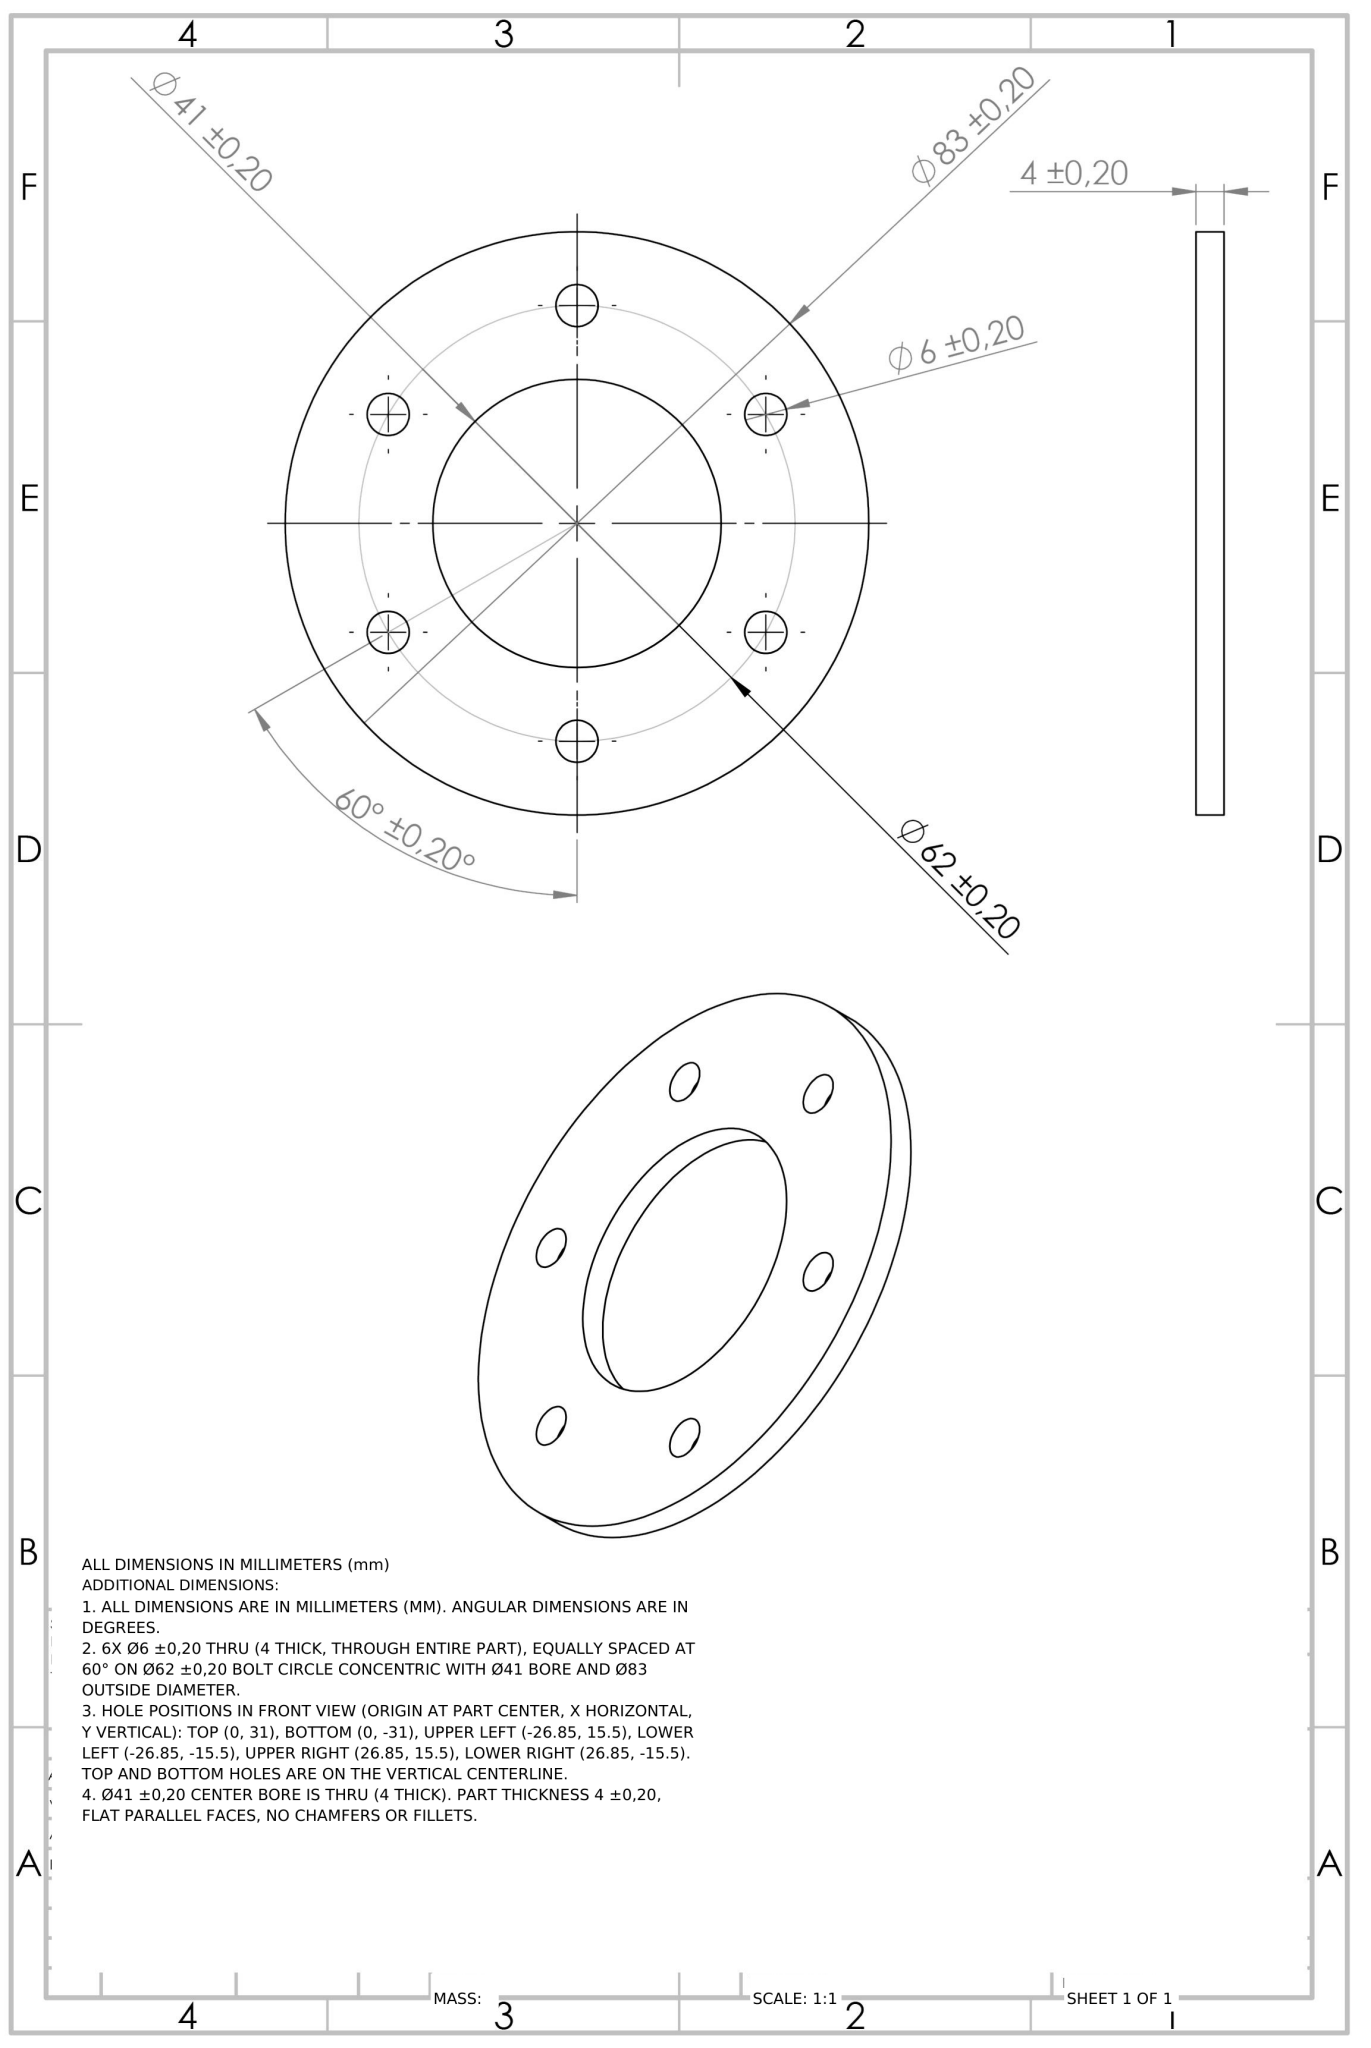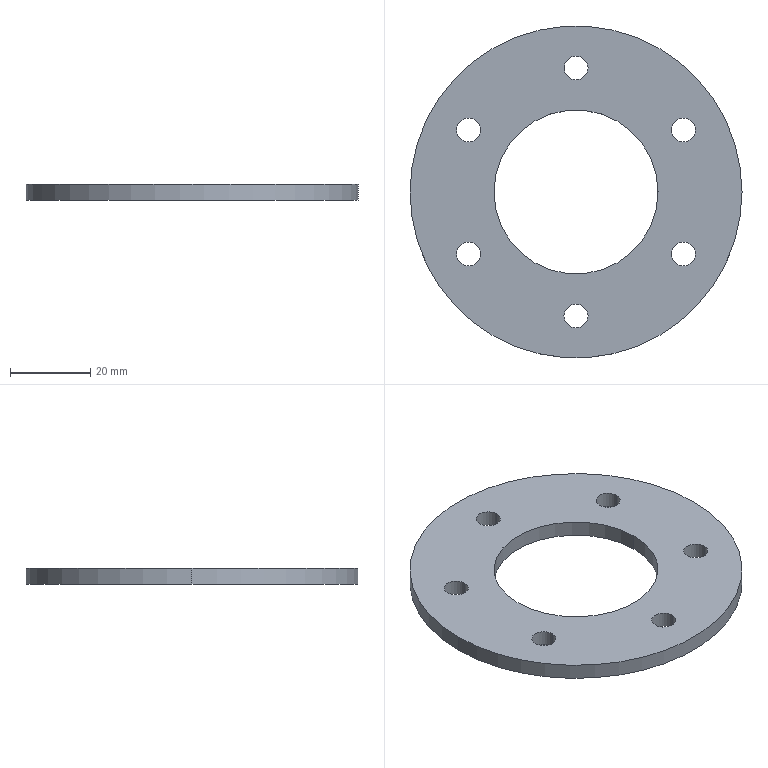Part | NX | mm | Six-Bolt Circular Flange Plate | 1 solid | 18 faces | box 83 x 83 x 4 mm | volume 15683 mm3 | cylinder 16 | plane 2 | commonest cylinder face diameters 6 x12 41 x2 83 x2
STEP:
#1=COLOUR_RGB('',0.7922,0.8196,0.9333);
#2=FILL_AREA_STYLE_COLOUR('',#1);
#3=FILL_AREA_STYLE('',(#2));
#4=SURFACE_STYLE_FILL_AREA(#3);
#5=SURFACE_SIDE_STYLE('',(#4));
#6=SURFACE_STYLE_USAGE(.BOTH.,#5);
#7=PRESENTATION_STYLE_ASSIGNMENT((#6));
#8=CARTESIAN_POINT('',(-29.847,15.5,4.));
#9=VERTEX_POINT('',#8);
#10=CARTESIAN_POINT('',(-23.847,15.5,4.));
#11=VERTEX_POINT('',#10);
#12=CARTESIAN_POINT('',(-26.847,15.5,4.));
#13=DIRECTION('',(0.,0.,1.));
#14=DIRECTION('',(1.,0.,0.));
#15=AXIS2_PLACEMENT_3D('',#12,#13,#14);
#16=CIRCLE('',#15,3.);
#17=EDGE_CURVE('',#9,#11,#16,.T.);
#18=ORIENTED_EDGE('',*,*,#17,.T.);
#19=CARTESIAN_POINT('',(-23.847,15.5,0.));
#20=VERTEX_POINT('',#19);
#21=CARTESIAN_POINT('',(-23.847,15.5,4.));
#22=DIRECTION('',(0.,0.,-1.));
#23=VECTOR('',#22,1000.);
#24=LINE('',#21,#23);
#25=EDGE_CURVE('',#11,#20,#24,.T.);
#26=ORIENTED_EDGE('',*,*,#25,.T.);
#27=CARTESIAN_POINT('',(-29.847,15.5,0.));
#28=VERTEX_POINT('',#27);
#29=CARTESIAN_POINT('',(-26.847,15.5,0.));
#30=DIRECTION('',(0.,0.,1.));
#31=DIRECTION('',(1.,0.,0.));
#32=AXIS2_PLACEMENT_3D('',#29,#30,#31);
#33=CIRCLE('',#32,3.);
#34=EDGE_CURVE('',#28,#20,#33,.T.);
#35=ORIENTED_EDGE('',*,*,#34,.F.);
#36=CARTESIAN_POINT('',(-29.847,15.5,4.));
#37=DIRECTION('',(0.,0.,-1.));
#38=VECTOR('',#37,1000.);
#39=LINE('',#36,#38);
#40=EDGE_CURVE('',#9,#28,#39,.T.);
#41=ORIENTED_EDGE('',*,*,#40,.F.);
#42=EDGE_LOOP('',(#18,#26,#35,#41));
#43=FACE_OUTER_BOUND('',#42,.T.);
#44=CARTESIAN_POINT('',(-26.847,15.5,4.));
#45=DIRECTION('',(0.,0.,-1.));
#46=DIRECTION('',(-1.,0.,0.));
#47=AXIS2_PLACEMENT_3D('',#44,#45,#46);
#48=CYLINDRICAL_SURFACE('',#47,3.);
#49=ADVANCED_FACE('',(#43),#48,.F.);
#50=CARTESIAN_POINT('',(-29.847,-15.5,4.));
#51=VERTEX_POINT('',#50);
#52=CARTESIAN_POINT('',(-23.847,-15.5,4.));
#53=VERTEX_POINT('',#52);
#54=CARTESIAN_POINT('',(-26.847,-15.5,4.));
#55=DIRECTION('',(0.,0.,1.));
#56=DIRECTION('',(1.,0.,0.));
#57=AXIS2_PLACEMENT_3D('',#54,#55,#56);
#58=CIRCLE('',#57,3.);
#59=EDGE_CURVE('',#51,#53,#58,.T.);
#60=ORIENTED_EDGE('',*,*,#59,.T.);
#61=CARTESIAN_POINT('',(-23.847,-15.5,0.));
#62=VERTEX_POINT('',#61);
#63=CARTESIAN_POINT('',(-23.847,-15.5,4.));
#64=DIRECTION('',(0.,0.,-1.));
#65=VECTOR('',#64,1000.);
#66=LINE('',#63,#65);
#67=EDGE_CURVE('',#53,#62,#66,.T.);
#68=ORIENTED_EDGE('',*,*,#67,.T.);
#69=CARTESIAN_POINT('',(-29.847,-15.5,0.));
#70=VERTEX_POINT('',#69);
#71=CARTESIAN_POINT('',(-26.847,-15.5,0.));
#72=DIRECTION('',(0.,0.,1.));
#73=DIRECTION('',(1.,0.,0.));
#74=AXIS2_PLACEMENT_3D('',#71,#72,#73);
#75=CIRCLE('',#74,3.);
#76=EDGE_CURVE('',#70,#62,#75,.T.);
#77=ORIENTED_EDGE('',*,*,#76,.F.);
#78=CARTESIAN_POINT('',(-29.847,-15.5,4.));
#79=DIRECTION('',(0.,0.,-1.));
#80=VECTOR('',#79,1000.);
#81=LINE('',#78,#80);
#82=EDGE_CURVE('',#51,#70,#81,.T.);
#83=ORIENTED_EDGE('',*,*,#82,.F.);
#84=EDGE_LOOP('',(#60,#68,#77,#83));
#85=FACE_OUTER_BOUND('',#84,.T.);
#86=CARTESIAN_POINT('',(-26.847,-15.5,4.));
#87=DIRECTION('',(0.,0.,-1.));
#88=DIRECTION('',(-1.,0.,0.));
#89=AXIS2_PLACEMENT_3D('',#86,#87,#88);
#90=CYLINDRICAL_SURFACE('',#89,3.);
#91=ADVANCED_FACE('',(#85),#90,.F.);
#92=CARTESIAN_POINT('',(-3.,-31.,4.));
#93=VERTEX_POINT('',#92);
#94=CARTESIAN_POINT('',(3.,-31.,4.));
#95=VERTEX_POINT('',#94);
#96=CARTESIAN_POINT('',(0.,-31.,4.));
#97=DIRECTION('',(0.,0.,1.));
#98=DIRECTION('',(1.,0.,0.));
#99=AXIS2_PLACEMENT_3D('',#96,#97,#98);
#100=CIRCLE('',#99,3.);
#101=EDGE_CURVE('',#93,#95,#100,.T.);
#102=ORIENTED_EDGE('',*,*,#101,.T.);
#103=CARTESIAN_POINT('',(3.,-31.,0.));
#104=VERTEX_POINT('',#103);
#105=CARTESIAN_POINT('',(3.,-31.,4.));
#106=DIRECTION('',(0.,0.,-1.));
#107=VECTOR('',#106,1000.);
#108=LINE('',#105,#107);
#109=EDGE_CURVE('',#95,#104,#108,.T.);
#110=ORIENTED_EDGE('',*,*,#109,.T.);
#111=CARTESIAN_POINT('',(-3.,-31.,0.));
#112=VERTEX_POINT('',#111);
#113=CARTESIAN_POINT('',(0.,-31.,0.));
#114=DIRECTION('',(0.,0.,1.));
#115=DIRECTION('',(1.,0.,0.));
#116=AXIS2_PLACEMENT_3D('',#113,#114,#115);
#117=CIRCLE('',#116,3.);
#118=EDGE_CURVE('',#112,#104,#117,.T.);
#119=ORIENTED_EDGE('',*,*,#118,.F.);
#120=CARTESIAN_POINT('',(-3.,-31.,4.));
#121=DIRECTION('',(0.,0.,-1.));
#122=VECTOR('',#121,1000.);
#123=LINE('',#120,#122);
#124=EDGE_CURVE('',#93,#112,#123,.T.);
#125=ORIENTED_EDGE('',*,*,#124,.F.);
#126=EDGE_LOOP('',(#102,#110,#119,#125));
#127=FACE_OUTER_BOUND('',#126,.T.);
#128=CARTESIAN_POINT('',(0.,-31.,4.));
#129=DIRECTION('',(0.,0.,-1.));
#130=DIRECTION('',(-1.,0.,0.));
#131=AXIS2_PLACEMENT_3D('',#128,#129,#130);
#132=CYLINDRICAL_SURFACE('',#131,3.);
#133=ADVANCED_FACE('',(#127),#132,.F.);
#134=CARTESIAN_POINT('',(23.847,-15.5,4.));
#135=VERTEX_POINT('',#134);
#136=CARTESIAN_POINT('',(29.847,-15.5,4.));
#137=VERTEX_POINT('',#136);
#138=CARTESIAN_POINT('',(26.847,-15.5,4.));
#139=DIRECTION('',(0.,0.,1.));
#140=DIRECTION('',(1.,0.,0.));
#141=AXIS2_PLACEMENT_3D('',#138,#139,#140);
#142=CIRCLE('',#141,3.);
#143=EDGE_CURVE('',#135,#137,#142,.T.);
#144=ORIENTED_EDGE('',*,*,#143,.T.);
#145=CARTESIAN_POINT('',(29.847,-15.5,0.));
#146=VERTEX_POINT('',#145);
#147=CARTESIAN_POINT('',(29.847,-15.5,4.));
#148=DIRECTION('',(0.,0.,-1.));
#149=VECTOR('',#148,1000.);
#150=LINE('',#147,#149);
#151=EDGE_CURVE('',#137,#146,#150,.T.);
#152=ORIENTED_EDGE('',*,*,#151,.T.);
#153=CARTESIAN_POINT('',(23.847,-15.5,0.));
#154=VERTEX_POINT('',#153);
#155=CARTESIAN_POINT('',(26.847,-15.5,0.));
#156=DIRECTION('',(0.,0.,1.));
#157=DIRECTION('',(1.,0.,0.));
#158=AXIS2_PLACEMENT_3D('',#155,#156,#157);
#159=CIRCLE('',#158,3.);
#160=EDGE_CURVE('',#154,#146,#159,.T.);
#161=ORIENTED_EDGE('',*,*,#160,.F.);
#162=CARTESIAN_POINT('',(23.847,-15.5,4.));
#163=DIRECTION('',(0.,0.,-1.));
#164=VECTOR('',#163,1000.);
#165=LINE('',#162,#164);
#166=EDGE_CURVE('',#135,#154,#165,.T.);
#167=ORIENTED_EDGE('',*,*,#166,.F.);
#168=EDGE_LOOP('',(#144,#152,#161,#167));
#169=FACE_OUTER_BOUND('',#168,.T.);
#170=CARTESIAN_POINT('',(26.847,-15.5,4.));
#171=DIRECTION('',(0.,0.,-1.));
#172=DIRECTION('',(-1.,0.,0.));
#173=AXIS2_PLACEMENT_3D('',#170,#171,#172);
#174=CYLINDRICAL_SURFACE('',#173,3.);
#175=ADVANCED_FACE('',(#169),#174,.F.);
#176=CARTESIAN_POINT('',(23.847,15.5,4.));
#177=VERTEX_POINT('',#176);
#178=CARTESIAN_POINT('',(29.847,15.5,4.));
#179=VERTEX_POINT('',#178);
#180=CARTESIAN_POINT('',(26.847,15.5,4.));
#181=DIRECTION('',(0.,0.,1.));
#182=DIRECTION('',(1.,0.,0.));
#183=AXIS2_PLACEMENT_3D('',#180,#181,#182);
#184=CIRCLE('',#183,3.);
#185=EDGE_CURVE('',#177,#179,#184,.T.);
#186=ORIENTED_EDGE('',*,*,#185,.T.);
#187=CARTESIAN_POINT('',(29.847,15.5,0.));
#188=VERTEX_POINT('',#187);
#189=CARTESIAN_POINT('',(29.847,15.5,4.));
#190=DIRECTION('',(0.,0.,-1.));
#191=VECTOR('',#190,1000.);
#192=LINE('',#189,#191);
#193=EDGE_CURVE('',#179,#188,#192,.T.);
#194=ORIENTED_EDGE('',*,*,#193,.T.);
#195=CARTESIAN_POINT('',(23.847,15.5,0.));
#196=VERTEX_POINT('',#195);
#197=CARTESIAN_POINT('',(26.847,15.5,0.));
#198=DIRECTION('',(0.,0.,1.));
#199=DIRECTION('',(1.,0.,0.));
#200=AXIS2_PLACEMENT_3D('',#197,#198,#199);
#201=CIRCLE('',#200,3.);
#202=EDGE_CURVE('',#196,#188,#201,.T.);
#203=ORIENTED_EDGE('',*,*,#202,.F.);
#204=CARTESIAN_POINT('',(23.847,15.5,4.));
#205=DIRECTION('',(0.,0.,-1.));
#206=VECTOR('',#205,1000.);
#207=LINE('',#204,#206);
#208=EDGE_CURVE('',#177,#196,#207,.T.);
#209=ORIENTED_EDGE('',*,*,#208,.F.);
#210=EDGE_LOOP('',(#186,#194,#203,#209));
#211=FACE_OUTER_BOUND('',#210,.T.);
#212=CARTESIAN_POINT('',(26.847,15.5,4.));
#213=DIRECTION('',(0.,0.,-1.));
#214=DIRECTION('',(-1.,0.,0.));
#215=AXIS2_PLACEMENT_3D('',#212,#213,#214);
#216=CYLINDRICAL_SURFACE('',#215,3.);
#217=ADVANCED_FACE('',(#211),#216,.F.);
#218=CARTESIAN_POINT('',(-3.,31.,4.));
#219=VERTEX_POINT('',#218);
#220=CARTESIAN_POINT('',(3.,31.,4.));
#221=VERTEX_POINT('',#220);
#222=CARTESIAN_POINT('',(0.,31.,4.));
#223=DIRECTION('',(0.,0.,1.));
#224=DIRECTION('',(1.,0.,0.));
#225=AXIS2_PLACEMENT_3D('',#222,#223,#224);
#226=CIRCLE('',#225,3.);
#227=EDGE_CURVE('',#219,#221,#226,.T.);
#228=ORIENTED_EDGE('',*,*,#227,.T.);
#229=CARTESIAN_POINT('',(3.,31.,0.));
#230=VERTEX_POINT('',#229);
#231=CARTESIAN_POINT('',(3.,31.,4.));
#232=DIRECTION('',(0.,0.,-1.));
#233=VECTOR('',#232,1000.);
#234=LINE('',#231,#233);
#235=EDGE_CURVE('',#221,#230,#234,.T.);
#236=ORIENTED_EDGE('',*,*,#235,.T.);
#237=CARTESIAN_POINT('',(-3.,31.,0.));
#238=VERTEX_POINT('',#237);
#239=CARTESIAN_POINT('',(0.,31.,0.));
#240=DIRECTION('',(0.,0.,1.));
#241=DIRECTION('',(1.,0.,0.));
#242=AXIS2_PLACEMENT_3D('',#239,#240,#241);
#243=CIRCLE('',#242,3.);
#244=EDGE_CURVE('',#238,#230,#243,.T.);
#245=ORIENTED_EDGE('',*,*,#244,.F.);
#246=CARTESIAN_POINT('',(-3.,31.,4.));
#247=DIRECTION('',(0.,0.,-1.));
#248=VECTOR('',#247,1000.);
#249=LINE('',#246,#248);
#250=EDGE_CURVE('',#219,#238,#249,.T.);
#251=ORIENTED_EDGE('',*,*,#250,.F.);
#252=EDGE_LOOP('',(#228,#236,#245,#251));
#253=FACE_OUTER_BOUND('',#252,.T.);
#254=CARTESIAN_POINT('',(0.,31.,4.));
#255=DIRECTION('',(0.,0.,-1.));
#256=DIRECTION('',(-1.,0.,0.));
#257=AXIS2_PLACEMENT_3D('',#254,#255,#256);
#258=CYLINDRICAL_SURFACE('',#257,3.);
#259=ADVANCED_FACE('',(#253),#258,.F.);
#260=CARTESIAN_POINT('',(-20.5,0.,4.));
#261=VERTEX_POINT('',#260);
#262=CARTESIAN_POINT('',(20.5,0.,4.));
#263=VERTEX_POINT('',#262);
#264=CARTESIAN_POINT('',(0.,0.,4.));
#265=DIRECTION('',(0.,0.,1.));
#266=DIRECTION('',(1.,0.,0.));
#267=AXIS2_PLACEMENT_3D('',#264,#265,#266);
#268=CIRCLE('',#267,20.5);
#269=EDGE_CURVE('',#261,#263,#268,.T.);
#270=ORIENTED_EDGE('',*,*,#269,.T.);
#271=CARTESIAN_POINT('',(20.5,0.,0.));
#272=VERTEX_POINT('',#271);
#273=CARTESIAN_POINT('',(20.5,0.,4.));
#274=DIRECTION('',(0.,0.,-1.));
#275=VECTOR('',#274,1000.);
#276=LINE('',#273,#275);
#277=EDGE_CURVE('',#263,#272,#276,.T.);
#278=ORIENTED_EDGE('',*,*,#277,.T.);
#279=CARTESIAN_POINT('',(-20.5,0.,0.));
#280=VERTEX_POINT('',#279);
#281=CARTESIAN_POINT('',(0.,0.,0.));
#282=DIRECTION('',(0.,0.,1.));
#283=DIRECTION('',(1.,0.,0.));
#284=AXIS2_PLACEMENT_3D('',#281,#282,#283);
#285=CIRCLE('',#284,20.5);
#286=EDGE_CURVE('',#280,#272,#285,.T.);
#287=ORIENTED_EDGE('',*,*,#286,.F.);
#288=CARTESIAN_POINT('',(-20.5,0.,4.));
#289=DIRECTION('',(0.,0.,-1.));
#290=VECTOR('',#289,1000.);
#291=LINE('',#288,#290);
#292=EDGE_CURVE('',#261,#280,#291,.T.);
#293=ORIENTED_EDGE('',*,*,#292,.F.);
#294=EDGE_LOOP('',(#270,#278,#287,#293));
#295=FACE_OUTER_BOUND('',#294,.T.);
#296=CARTESIAN_POINT('',(0.,0.,4.));
#297=DIRECTION('',(0.,0.,-1.));
#298=DIRECTION('',(-1.,0.,0.));
#299=AXIS2_PLACEMENT_3D('',#296,#297,#298);
#300=CYLINDRICAL_SURFACE('',#299,20.5);
#301=ADVANCED_FACE('',(#295),#300,.F.);
#302=CARTESIAN_POINT('',(41.5,0.,4.));
#303=VERTEX_POINT('',#302);
#304=CARTESIAN_POINT('',(-41.5,0.,4.));
#305=VERTEX_POINT('',#304);
#306=CARTESIAN_POINT('',(0.,0.,4.));
#307=DIRECTION('',(0.,0.,1.));
#308=DIRECTION('',(1.,0.,0.));
#309=AXIS2_PLACEMENT_3D('',#306,#307,#308);
#310=CIRCLE('',#309,41.5);
#311=EDGE_CURVE('',#303,#305,#310,.T.);
#312=ORIENTED_EDGE('',*,*,#311,.F.);
#313=CARTESIAN_POINT('',(41.5,0.,0.));
#314=VERTEX_POINT('',#313);
#315=CARTESIAN_POINT('',(41.5,0.,4.));
#316=DIRECTION('',(0.,0.,-1.));
#317=VECTOR('',#316,1000.);
#318=LINE('',#315,#317);
#319=EDGE_CURVE('',#303,#314,#318,.T.);
#320=ORIENTED_EDGE('',*,*,#319,.T.);
#321=CARTESIAN_POINT('',(-41.5,0.,0.));
#322=VERTEX_POINT('',#321);
#323=CARTESIAN_POINT('',(0.,0.,0.));
#324=DIRECTION('',(0.,0.,1.));
#325=DIRECTION('',(1.,0.,0.));
#326=AXIS2_PLACEMENT_3D('',#323,#324,#325);
#327=CIRCLE('',#326,41.5);
#328=EDGE_CURVE('',#314,#322,#327,.T.);
#329=ORIENTED_EDGE('',*,*,#328,.T.);
#330=CARTESIAN_POINT('',(-41.5,0.,4.));
#331=DIRECTION('',(0.,0.,-1.));
#332=VECTOR('',#331,1000.);
#333=LINE('',#330,#332);
#334=EDGE_CURVE('',#305,#322,#333,.T.);
#335=ORIENTED_EDGE('',*,*,#334,.F.);
#336=EDGE_LOOP('',(#312,#320,#329,#335));
#337=FACE_OUTER_BOUND('',#336,.T.);
#338=CARTESIAN_POINT('',(0.,0.,4.));
#339=DIRECTION('',(0.,0.,-1.));
#340=DIRECTION('',(-1.,0.,0.));
#341=AXIS2_PLACEMENT_3D('',#338,#339,#340);
#342=CYLINDRICAL_SURFACE('',#341,41.5);
#343=ADVANCED_FACE('',(#337),#342,.T.);
#344=ORIENTED_EDGE('',*,*,#59,.F.);
#345=CARTESIAN_POINT('',(-26.847,-15.5,4.));
#346=DIRECTION('',(0.,0.,1.));
#347=DIRECTION('',(1.,0.,0.));
#348=AXIS2_PLACEMENT_3D('',#345,#346,#347);
#349=CIRCLE('',#348,3.);
#350=EDGE_CURVE('',#53,#51,#349,.T.);
#351=ORIENTED_EDGE('',*,*,#350,.F.);
#352=EDGE_LOOP('',(#344,#351));
#353=FACE_BOUND('',#352,.T.);
#354=ORIENTED_EDGE('',*,*,#143,.F.);
#355=CARTESIAN_POINT('',(26.847,-15.5,4.));
#356=DIRECTION('',(0.,0.,1.));
#357=DIRECTION('',(1.,0.,0.));
#358=AXIS2_PLACEMENT_3D('',#355,#356,#357);
#359=CIRCLE('',#358,3.);
#360=EDGE_CURVE('',#137,#135,#359,.T.);
#361=ORIENTED_EDGE('',*,*,#360,.F.);
#362=EDGE_LOOP('',(#354,#361));
#363=FACE_BOUND('',#362,.T.);
#364=ORIENTED_EDGE('',*,*,#227,.F.);
#365=CARTESIAN_POINT('',(0.,31.,4.));
#366=DIRECTION('',(0.,0.,1.));
#367=DIRECTION('',(1.,0.,0.));
#368=AXIS2_PLACEMENT_3D('',#365,#366,#367);
#369=CIRCLE('',#368,3.);
#370=EDGE_CURVE('',#221,#219,#369,.T.);
#371=ORIENTED_EDGE('',*,*,#370,.F.);
#372=EDGE_LOOP('',(#364,#371));
#373=FACE_BOUND('',#372,.T.);
#374=CARTESIAN_POINT('',(0.,0.,4.));
#375=DIRECTION('',(0.,0.,1.));
#376=DIRECTION('',(1.,0.,0.));
#377=AXIS2_PLACEMENT_3D('',#374,#375,#376);
#378=CIRCLE('',#377,41.5);
#379=EDGE_CURVE('',#305,#303,#378,.T.);
#380=ORIENTED_EDGE('',*,*,#379,.T.);
#381=ORIENTED_EDGE('',*,*,#311,.T.);
#382=EDGE_LOOP('',(#380,#381));
#383=FACE_OUTER_BOUND('',#382,.T.);
#384=ORIENTED_EDGE('',*,*,#269,.F.);
#385=CARTESIAN_POINT('',(0.,0.,4.));
#386=DIRECTION('',(0.,0.,1.));
#387=DIRECTION('',(1.,0.,0.));
#388=AXIS2_PLACEMENT_3D('',#385,#386,#387);
#389=CIRCLE('',#388,20.5);
#390=EDGE_CURVE('',#263,#261,#389,.T.);
#391=ORIENTED_EDGE('',*,*,#390,.F.);
#392=EDGE_LOOP('',(#384,#391));
#393=FACE_BOUND('',#392,.T.);
#394=ORIENTED_EDGE('',*,*,#185,.F.);
#395=CARTESIAN_POINT('',(26.847,15.5,4.));
#396=DIRECTION('',(0.,0.,1.));
#397=DIRECTION('',(1.,0.,0.));
#398=AXIS2_PLACEMENT_3D('',#395,#396,#397);
#399=CIRCLE('',#398,3.);
#400=EDGE_CURVE('',#179,#177,#399,.T.);
#401=ORIENTED_EDGE('',*,*,#400,.F.);
#402=EDGE_LOOP('',(#394,#401));
#403=FACE_BOUND('',#402,.T.);
#404=ORIENTED_EDGE('',*,*,#101,.F.);
#405=CARTESIAN_POINT('',(0.,-31.,4.));
#406=DIRECTION('',(0.,0.,1.));
#407=DIRECTION('',(1.,0.,0.));
#408=AXIS2_PLACEMENT_3D('',#405,#406,#407);
#409=CIRCLE('',#408,3.);
#410=EDGE_CURVE('',#95,#93,#409,.T.);
#411=ORIENTED_EDGE('',*,*,#410,.F.);
#412=EDGE_LOOP('',(#404,#411));
#413=FACE_BOUND('',#412,.T.);
#414=ORIENTED_EDGE('',*,*,#17,.F.);
#415=CARTESIAN_POINT('',(-26.847,15.5,4.));
#416=DIRECTION('',(0.,0.,1.));
#417=DIRECTION('',(1.,0.,0.));
#418=AXIS2_PLACEMENT_3D('',#415,#416,#417);
#419=CIRCLE('',#418,3.);
#420=EDGE_CURVE('',#11,#9,#419,.T.);
#421=ORIENTED_EDGE('',*,*,#420,.F.);
#422=EDGE_LOOP('',(#414,#421));
#423=FACE_BOUND('',#422,.T.);
#424=CARTESIAN_POINT('',(0.,0.,4.));
#425=DIRECTION('',(0.,0.,1.));
#426=DIRECTION('',(1.,0.,0.));
#427=AXIS2_PLACEMENT_3D('',#424,#425,#426);
#428=PLANE('',#427);
#429=ADVANCED_FACE('',(#353,#363,#373,#383,#393,#403,#413,#423),#428,.T.);
#430=CARTESIAN_POINT('',(0.,0.,0.));
#431=DIRECTION('',(0.,0.,1.));
#432=DIRECTION('',(1.,0.,0.));
#433=AXIS2_PLACEMENT_3D('',#430,#431,#432);
#434=CIRCLE('',#433,41.5);
#435=EDGE_CURVE('',#322,#314,#434,.T.);
#436=ORIENTED_EDGE('',*,*,#435,.F.);
#437=ORIENTED_EDGE('',*,*,#328,.F.);
#438=EDGE_LOOP('',(#436,#437));
#439=FACE_OUTER_BOUND('',#438,.T.);
#440=ORIENTED_EDGE('',*,*,#286,.T.);
#441=CARTESIAN_POINT('',(0.,0.,0.));
#442=DIRECTION('',(0.,0.,1.));
#443=DIRECTION('',(1.,0.,0.));
#444=AXIS2_PLACEMENT_3D('',#441,#442,#443);
#445=CIRCLE('',#444,20.5);
#446=EDGE_CURVE('',#272,#280,#445,.T.);
#447=ORIENTED_EDGE('',*,*,#446,.T.);
#448=EDGE_LOOP('',(#440,#447));
#449=FACE_BOUND('',#448,.T.);
#450=ORIENTED_EDGE('',*,*,#244,.T.);
#451=CARTESIAN_POINT('',(0.,31.,0.));
#452=DIRECTION('',(0.,0.,1.));
#453=DIRECTION('',(1.,0.,0.));
#454=AXIS2_PLACEMENT_3D('',#451,#452,#453);
#455=CIRCLE('',#454,3.);
#456=EDGE_CURVE('',#230,#238,#455,.T.);
#457=ORIENTED_EDGE('',*,*,#456,.T.);
#458=EDGE_LOOP('',(#450,#457));
#459=FACE_BOUND('',#458,.T.);
#460=ORIENTED_EDGE('',*,*,#202,.T.);
#461=CARTESIAN_POINT('',(26.847,15.5,0.));
#462=DIRECTION('',(0.,0.,1.));
#463=DIRECTION('',(1.,0.,0.));
#464=AXIS2_PLACEMENT_3D('',#461,#462,#463);
#465=CIRCLE('',#464,3.);
#466=EDGE_CURVE('',#188,#196,#465,.T.);
#467=ORIENTED_EDGE('',*,*,#466,.T.);
#468=EDGE_LOOP('',(#460,#467));
#469=FACE_BOUND('',#468,.T.);
#470=ORIENTED_EDGE('',*,*,#160,.T.);
#471=CARTESIAN_POINT('',(26.847,-15.5,0.));
#472=DIRECTION('',(0.,0.,1.));
#473=DIRECTION('',(1.,0.,0.));
#474=AXIS2_PLACEMENT_3D('',#471,#472,#473);
#475=CIRCLE('',#474,3.);
#476=EDGE_CURVE('',#146,#154,#475,.T.);
#477=ORIENTED_EDGE('',*,*,#476,.T.);
#478=EDGE_LOOP('',(#470,#477));
#479=FACE_BOUND('',#478,.T.);
#480=ORIENTED_EDGE('',*,*,#118,.T.);
#481=CARTESIAN_POINT('',(0.,-31.,0.));
#482=DIRECTION('',(0.,0.,1.));
#483=DIRECTION('',(1.,0.,0.));
#484=AXIS2_PLACEMENT_3D('',#481,#482,#483);
#485=CIRCLE('',#484,3.);
#486=EDGE_CURVE('',#104,#112,#485,.T.);
#487=ORIENTED_EDGE('',*,*,#486,.T.);
#488=EDGE_LOOP('',(#480,#487));
#489=FACE_BOUND('',#488,.T.);
#490=ORIENTED_EDGE('',*,*,#76,.T.);
#491=CARTESIAN_POINT('',(-26.847,-15.5,0.));
#492=DIRECTION('',(0.,0.,1.));
#493=DIRECTION('',(1.,0.,0.));
#494=AXIS2_PLACEMENT_3D('',#491,#492,#493);
#495=CIRCLE('',#494,3.);
#496=EDGE_CURVE('',#62,#70,#495,.T.);
#497=ORIENTED_EDGE('',*,*,#496,.T.);
#498=EDGE_LOOP('',(#490,#497));
#499=FACE_BOUND('',#498,.T.);
#500=ORIENTED_EDGE('',*,*,#34,.T.);
#501=CARTESIAN_POINT('',(-26.847,15.5,0.));
#502=DIRECTION('',(0.,0.,1.));
#503=DIRECTION('',(1.,0.,0.));
#504=AXIS2_PLACEMENT_3D('',#501,#502,#503);
#505=CIRCLE('',#504,3.);
#506=EDGE_CURVE('',#20,#28,#505,.T.);
#507=ORIENTED_EDGE('',*,*,#506,.T.);
#508=EDGE_LOOP('',(#500,#507));
#509=FACE_BOUND('',#508,.T.);
#510=CARTESIAN_POINT('',(0.,0.,0.));
#511=DIRECTION('',(0.,0.,1.));
#512=DIRECTION('',(1.,0.,0.));
#513=AXIS2_PLACEMENT_3D('',#510,#511,#512);
#514=PLANE('',#513);
#515=ADVANCED_FACE('',(#439,#449,#459,#469,#479,#489,#499,#509),#514,.F.);
#516=ORIENTED_EDGE('',*,*,#319,.F.);
#517=ORIENTED_EDGE('',*,*,#379,.F.);
#518=ORIENTED_EDGE('',*,*,#334,.T.);
#519=ORIENTED_EDGE('',*,*,#435,.T.);
#520=EDGE_LOOP('',(#516,#517,#518,#519));
#521=FACE_OUTER_BOUND('',#520,.T.);
#522=CARTESIAN_POINT('',(0.,0.,4.));
#523=DIRECTION('',(0.,0.,-1.));
#524=DIRECTION('',(-1.,0.,0.));
#525=AXIS2_PLACEMENT_3D('',#522,#523,#524);
#526=CYLINDRICAL_SURFACE('',#525,41.5);
#527=ADVANCED_FACE('',(#521),#526,.T.);
#528=ORIENTED_EDGE('',*,*,#277,.F.);
#529=ORIENTED_EDGE('',*,*,#390,.T.);
#530=ORIENTED_EDGE('',*,*,#292,.T.);
#531=ORIENTED_EDGE('',*,*,#446,.F.);
#532=EDGE_LOOP('',(#528,#529,#530,#531));
#533=FACE_OUTER_BOUND('',#532,.T.);
#534=CARTESIAN_POINT('',(0.,0.,4.));
#535=DIRECTION('',(0.,0.,-1.));
#536=DIRECTION('',(-1.,0.,0.));
#537=AXIS2_PLACEMENT_3D('',#534,#535,#536);
#538=CYLINDRICAL_SURFACE('',#537,20.5);
#539=ADVANCED_FACE('',(#533),#538,.F.);
#540=ORIENTED_EDGE('',*,*,#235,.F.);
#541=ORIENTED_EDGE('',*,*,#370,.T.);
#542=ORIENTED_EDGE('',*,*,#250,.T.);
#543=ORIENTED_EDGE('',*,*,#456,.F.);
#544=EDGE_LOOP('',(#540,#541,#542,#543));
#545=FACE_OUTER_BOUND('',#544,.T.);
#546=CARTESIAN_POINT('',(0.,31.,4.));
#547=DIRECTION('',(0.,0.,-1.));
#548=DIRECTION('',(-1.,0.,0.));
#549=AXIS2_PLACEMENT_3D('',#546,#547,#548);
#550=CYLINDRICAL_SURFACE('',#549,3.);
#551=ADVANCED_FACE('',(#545),#550,.F.);
#552=ORIENTED_EDGE('',*,*,#193,.F.);
#553=ORIENTED_EDGE('',*,*,#400,.T.);
#554=ORIENTED_EDGE('',*,*,#208,.T.);
#555=ORIENTED_EDGE('',*,*,#466,.F.);
#556=EDGE_LOOP('',(#552,#553,#554,#555));
#557=FACE_OUTER_BOUND('',#556,.T.);
#558=CARTESIAN_POINT('',(26.847,15.5,4.));
#559=DIRECTION('',(0.,0.,-1.));
#560=DIRECTION('',(-1.,0.,0.));
#561=AXIS2_PLACEMENT_3D('',#558,#559,#560);
#562=CYLINDRICAL_SURFACE('',#561,3.);
#563=ADVANCED_FACE('',(#557),#562,.F.);
#564=ORIENTED_EDGE('',*,*,#151,.F.);
#565=ORIENTED_EDGE('',*,*,#360,.T.);
#566=ORIENTED_EDGE('',*,*,#166,.T.);
#567=ORIENTED_EDGE('',*,*,#476,.F.);
#568=EDGE_LOOP('',(#564,#565,#566,#567));
#569=FACE_OUTER_BOUND('',#568,.T.);
#570=CARTESIAN_POINT('',(26.847,-15.5,4.));
#571=DIRECTION('',(0.,0.,-1.));
#572=DIRECTION('',(-1.,0.,0.));
#573=AXIS2_PLACEMENT_3D('',#570,#571,#572);
#574=CYLINDRICAL_SURFACE('',#573,3.);
#575=ADVANCED_FACE('',(#569),#574,.F.);
#576=ORIENTED_EDGE('',*,*,#109,.F.);
#577=ORIENTED_EDGE('',*,*,#410,.T.);
#578=ORIENTED_EDGE('',*,*,#124,.T.);
#579=ORIENTED_EDGE('',*,*,#486,.F.);
#580=EDGE_LOOP('',(#576,#577,#578,#579));
#581=FACE_OUTER_BOUND('',#580,.T.);
#582=CARTESIAN_POINT('',(0.,-31.,4.));
#583=DIRECTION('',(0.,0.,-1.));
#584=DIRECTION('',(-1.,0.,0.));
#585=AXIS2_PLACEMENT_3D('',#582,#583,#584);
#586=CYLINDRICAL_SURFACE('',#585,3.);
#587=ADVANCED_FACE('',(#581),#586,.F.);
#588=ORIENTED_EDGE('',*,*,#67,.F.);
#589=ORIENTED_EDGE('',*,*,#350,.T.);
#590=ORIENTED_EDGE('',*,*,#82,.T.);
#591=ORIENTED_EDGE('',*,*,#496,.F.);
#592=EDGE_LOOP('',(#588,#589,#590,#591));
#593=FACE_OUTER_BOUND('',#592,.T.);
#594=CARTESIAN_POINT('',(-26.847,-15.5,4.));
#595=DIRECTION('',(0.,0.,-1.));
#596=DIRECTION('',(-1.,0.,0.));
#597=AXIS2_PLACEMENT_3D('',#594,#595,#596);
#598=CYLINDRICAL_SURFACE('',#597,3.);
#599=ADVANCED_FACE('',(#593),#598,.F.);
#600=ORIENTED_EDGE('',*,*,#25,.F.);
#601=ORIENTED_EDGE('',*,*,#420,.T.);
#602=ORIENTED_EDGE('',*,*,#40,.T.);
#603=ORIENTED_EDGE('',*,*,#506,.F.);
#604=EDGE_LOOP('',(#600,#601,#602,#603));
#605=FACE_OUTER_BOUND('',#604,.T.);
#606=CARTESIAN_POINT('',(-26.847,15.5,4.));
#607=DIRECTION('',(0.,0.,-1.));
#608=DIRECTION('',(-1.,0.,0.));
#609=AXIS2_PLACEMENT_3D('',#606,#607,#608);
#610=CYLINDRICAL_SURFACE('',#609,3.);
#611=ADVANCED_FACE('',(#605),#610,.F.);
#612=CLOSED_SHELL('',(#49,#91,#133,#175,#217,#259,#301,#343,#429,#515,#527,#539,#551,#563,#575,#587,#599,#611));
#613=MANIFOLD_SOLID_BREP('',#612);
#614=CARTESIAN_POINT('',(0.,0.,0.));
#615=DIRECTION('',(0.,0.,1.));
#616=DIRECTION('',(1.,0.,0.));
#617=AXIS2_PLACEMENT_3D('',#614,#615,#616);
#618=(LENGTH_UNIT()NAMED_UNIT(*)SI_UNIT(.MILLI.,.METRE.));
#619=UNCERTAINTY_MEASURE_WITH_UNIT(LENGTH_MEASURE(0.00001),#618,'','');
#620=(NAMED_UNIT(*)PLANE_ANGLE_UNIT()SI_UNIT($,.RADIAN.));
#621=(NAMED_UNIT(*)SI_UNIT($,.STERADIAN.)SOLID_ANGLE_UNIT());
#622=(GEOMETRIC_REPRESENTATION_CONTEXT(3)GLOBAL_UNCERTAINTY_ASSIGNED_CONTEXT((#619))GLOBAL_UNIT_ASSIGNED_CONTEXT((#618,#620,#621))REPRESENTATION_CONTEXT('',''));
#623=ADVANCED_BREP_SHAPE_REPRESENTATION('',(#613,#617),#622);
#624=STYLED_ITEM('',(#7),#623);
#625=(LENGTH_UNIT()NAMED_UNIT(*)SI_UNIT(.MILLI.,.METRE.));
#626=UNCERTAINTY_MEASURE_WITH_UNIT(LENGTH_MEASURE(0.00001),#625,'','');
#627=(NAMED_UNIT(*)PLANE_ANGLE_UNIT()SI_UNIT($,.RADIAN.));
#628=(NAMED_UNIT(*)SI_UNIT($,.STERADIAN.)SOLID_ANGLE_UNIT());
#629=(GEOMETRIC_REPRESENTATION_CONTEXT(3)GLOBAL_UNCERTAINTY_ASSIGNED_CONTEXT((#626))GLOBAL_UNIT_ASSIGNED_CONTEXT((#625,#627,#628))REPRESENTATION_CONTEXT('',''));
#630=MECHANICAL_DESIGN_GEOMETRIC_PRESENTATION_REPRESENTATION('',(#624),#629);
#631=COLOUR_RGB('',0.7922,0.8196,0.9333);
#632=FILL_AREA_STYLE_COLOUR('',#631);
#633=FILL_AREA_STYLE('',(#632));
#634=SURFACE_STYLE_FILL_AREA(#633);
#635=SURFACE_SIDE_STYLE('',(#634));
#636=SURFACE_STYLE_USAGE(.BOTH.,#635);
#637=PRESENTATION_STYLE_ASSIGNMENT((#636));
#638=STYLED_ITEM('',(#637),#613);
#639=PRESENTATION_LAYER_ASSIGNMENT('','',(#638));
#640=PRESENTATION_LAYER_ASSIGNMENT('','',(#624));
#641=(LENGTH_UNIT()NAMED_UNIT(*)SI_UNIT(.MILLI.,.METRE.));
#642=UNCERTAINTY_MEASURE_WITH_UNIT(LENGTH_MEASURE(0.00001),#641,'','');
#643=(NAMED_UNIT(*)PLANE_ANGLE_UNIT()SI_UNIT($,.RADIAN.));
#644=(NAMED_UNIT(*)SI_UNIT($,.STERADIAN.)SOLID_ANGLE_UNIT());
#645=(GEOMETRIC_REPRESENTATION_CONTEXT(3)GLOBAL_UNCERTAINTY_ASSIGNED_CONTEXT((#642))GLOBAL_UNIT_ASSIGNED_CONTEXT((#641,#643,#644))REPRESENTATION_CONTEXT('',''));
#646=MECHANICAL_DESIGN_GEOMETRIC_PRESENTATION_REPRESENTATION('',(#638),#645);